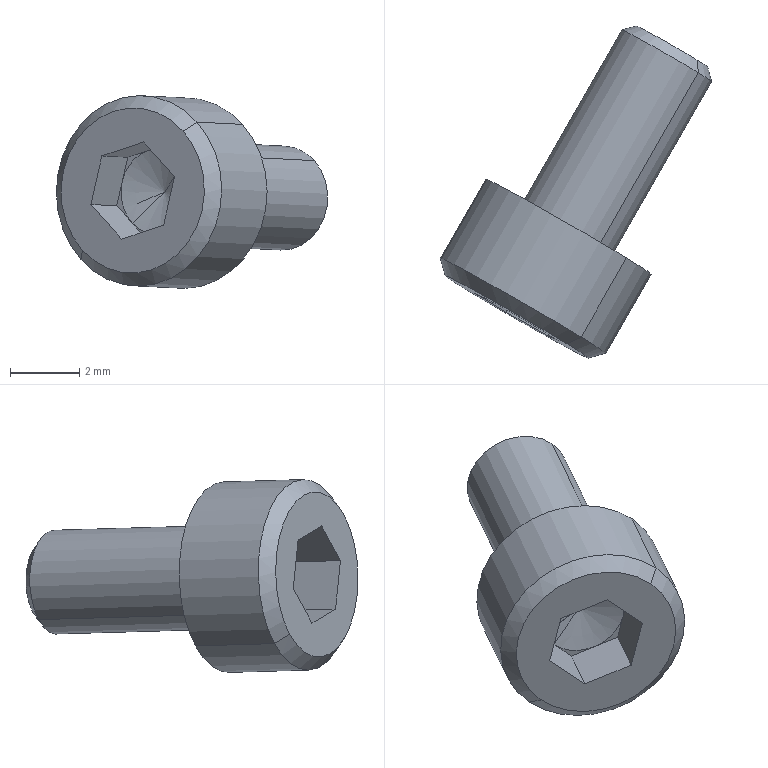Component | SolidWorks | KKSwitch-0710z0-123-1_CB3-6-0710z0-123-14 | 1 solid | 25 faces | box 7.83 x 9.58 x 5.56 mm | volume 103 mm3 | plane 15 | cone 6 | cylinder 4 | commonest cylinder face diameters 3 x2 5.5 x2
STEP:
#1=COLOUR_RGB('',0.7922,0.8196,0.9333);
#2=FILL_AREA_STYLE_COLOUR('',#1);
#3=FILL_AREA_STYLE('',(#2));
#4=SURFACE_STYLE_FILL_AREA(#3);
#5=SURFACE_SIDE_STYLE('',(#4));
#6=SURFACE_STYLE_USAGE(.BOTH.,#5);
#7=PRESENTATION_STYLE_ASSIGNMENT((#6));
#8=CARTESIAN_POINT('',(3.361,-1.018,8.462));
#9=VERTEX_POINT('',#8);
#10=CARTESIAN_POINT('',(3.433,-1.057,8.547));
#11=VERTEX_POINT('',#10);
#12=CARTESIAN_POINT('',(3.397,-1.037,8.504));
#13=DIRECTION('',(0.4977,0.867,-0.02519));
#14=DIRECTION('',(-0.6092,0.3288,-0.7216));
#15=AXIS2_PLACEMENT_3D('',#12,#13,#14);
#16=CIRCLE('',#15,0.05906);
#17=EDGE_CURVE('',#9,#11,#16,.T.);
#18=ORIENTED_EDGE('',*,*,#17,.T.);
#19=CARTESIAN_POINT('',(3.545,-0.8624,8.541));
#20=VERTEX_POINT('',#19);
#21=CARTESIAN_POINT('',(3.489,-0.9595,8.544));
#22=DIRECTION('',(0.4977,0.867,-0.02519));
#23=VECTOR('',#22,39.37);
#24=LINE('',#21,#23);
#25=EDGE_CURVE('',#11,#20,#24,.T.);
#26=ORIENTED_EDGE('',*,*,#25,.T.);
#27=CARTESIAN_POINT('',(3.473,-0.8236,8.456));
#28=VERTEX_POINT('',#27);
#29=CARTESIAN_POINT('',(3.509,-0.843,8.499));
#30=DIRECTION('',(-0.4977,-0.867,0.02519));
#31=DIRECTION('',(-0.6092,0.3288,-0.7216));
#32=AXIS2_PLACEMENT_3D('',#29,#30,#31);
#33=CIRCLE('',#32,0.05906);
#34=EDGE_CURVE('',#20,#28,#33,.T.);
#35=ORIENTED_EDGE('',*,*,#34,.T.);
#36=CARTESIAN_POINT('',(3.417,-0.9207,8.459));
#37=DIRECTION('',(0.4977,0.867,-0.02519));
#38=VECTOR('',#37,39.37);
#39=LINE('',#36,#38);
#40=EDGE_CURVE('',#9,#28,#39,.T.);
#41=ORIENTED_EDGE('',*,*,#40,.F.);
#42=EDGE_LOOP('',(#18,#26,#35,#41));
#43=FACE_OUTER_BOUND('',#42,.T.);
#44=CARTESIAN_POINT('',(3.453,-0.9401,8.501));
#45=DIRECTION('',(0.4977,0.867,-0.02519));
#46=DIRECTION('',(-0.6092,0.3288,-0.7216));
#47=AXIS2_PLACEMENT_3D('',#44,#45,#46);
#48=CYLINDRICAL_SURFACE('',#47,0.05906);
#49=ADVANCED_FACE('',(#43),#48,.T.);
#50=CARTESIAN_POINT('',(3.543,-0.8479,8.532));
#51=VERTEX_POINT('',#50);
#52=CARTESIAN_POINT('',(3.486,-0.817,8.464));
#53=VERTEX_POINT('',#52);
#54=CARTESIAN_POINT('',(3.515,-0.8325,8.498));
#55=DIRECTION('',(-0.4977,-0.867,0.02519));
#56=DIRECTION('',(0.6092,-0.3288,0.7216));
#57=AXIS2_PLACEMENT_3D('',#54,#55,#56);
#58=CIRCLE('',#57,0.04696);
#59=EDGE_CURVE('',#51,#53,#58,.T.);
#60=ORIENTED_EDGE('',*,*,#59,.T.);
#61=CARTESIAN_POINT('',(3.473,-0.8236,8.456));
#62=DIRECTION('',(-0.7827,-0.3806,-0.4924));
#63=VECTOR('',#62,39.37);
#64=LINE('',#61,#63);
#65=EDGE_CURVE('',#53,#28,#64,.T.);
#66=ORIENTED_EDGE('',*,*,#65,.T.);
#67=ORIENTED_EDGE('',*,*,#34,.F.);
#68=CARTESIAN_POINT('',(3.545,-0.8624,8.541));
#69=DIRECTION('',(0.07887,-0.8455,0.5281));
#70=VECTOR('',#69,39.37);
#71=LINE('',#68,#70);
#72=EDGE_CURVE('',#51,#20,#71,.T.);
#73=ORIENTED_EDGE('',*,*,#72,.F.);
#74=EDGE_LOOP('',(#60,#66,#67,#73));
#75=FACE_OUTER_BOUND('',#74,.T.);
#76=CARTESIAN_POINT('',(3.509,-0.843,8.499));
#77=DIRECTION('',(-0.4977,-0.867,0.02519));
#78=DIRECTION('',(0.6092,-0.3288,0.7216));
#79=AXIS2_PLACEMENT_3D('',#76,#77,#78);
#80=CONICAL_SURFACE('',#79,0.05906,0.7854);
#81=ADVANCED_FACE('',(#75),#80,.T.);
#82=CARTESIAN_POINT('',(3.279,-1.092,8.429));
#83=VERTEX_POINT('',#82);
#84=CARTESIAN_POINT('',(3.411,-1.163,8.585));
#85=VERTEX_POINT('',#84);
#86=CARTESIAN_POINT('',(3.345,-1.127,8.507));
#87=DIRECTION('',(0.4977,0.867,-0.02519));
#88=DIRECTION('',(-0.6092,0.3288,-0.7216));
#89=AXIS2_PLACEMENT_3D('',#86,#87,#88);
#90=CIRCLE('',#89,0.1083);
#91=EDGE_CURVE('',#83,#85,#90,.T.);
#92=ORIENTED_EDGE('',*,*,#91,.T.);
#93=CARTESIAN_POINT('',(3.463,-1.073,8.582));
#94=VERTEX_POINT('',#93);
#95=CARTESIAN_POINT('',(3.437,-1.118,8.584));
#96=DIRECTION('',(0.4977,0.867,-0.02519));
#97=VECTOR('',#96,39.37);
#98=LINE('',#95,#97);
#99=EDGE_CURVE('',#85,#94,#98,.T.);
#100=ORIENTED_EDGE('',*,*,#99,.T.);
#101=CARTESIAN_POINT('',(3.331,-1.002,8.426));
#102=VERTEX_POINT('',#101);
#103=CARTESIAN_POINT('',(3.397,-1.037,8.504));
#104=DIRECTION('',(0.4977,0.867,-0.02519));
#105=DIRECTION('',(-0.6092,0.3288,-0.7216));
#106=AXIS2_PLACEMENT_3D('',#103,#104,#105);
#107=CIRCLE('',#106,0.1083);
#108=EDGE_CURVE('',#102,#94,#107,.T.);
#109=ORIENTED_EDGE('',*,*,#108,.F.);
#110=CARTESIAN_POINT('',(3.305,-1.047,8.427));
#111=DIRECTION('',(0.4977,0.867,-0.02519));
#112=VECTOR('',#111,39.37);
#113=LINE('',#110,#112);
#114=EDGE_CURVE('',#83,#102,#113,.T.);
#115=ORIENTED_EDGE('',*,*,#114,.F.);
#116=EDGE_LOOP('',(#92,#100,#109,#115));
#117=FACE_OUTER_BOUND('',#116,.T.);
#118=CARTESIAN_POINT('',(3.371,-1.082,8.505));
#119=DIRECTION('',(0.4977,0.867,-0.02519));
#120=DIRECTION('',(-0.6092,0.3288,-0.7216));
#121=AXIS2_PLACEMENT_3D('',#118,#119,#120);
#122=CYLINDRICAL_SURFACE('',#121,0.1083);
#123=ADVANCED_FACE('',(#117),#122,.T.);
#124=CARTESIAN_POINT('',(3.281,-1.109,8.439));
#125=VERTEX_POINT('',#124);
#126=CARTESIAN_POINT('',(3.395,-1.171,8.575));
#127=VERTEX_POINT('',#126);
#128=CARTESIAN_POINT('',(3.338,-1.14,8.507));
#129=DIRECTION('',(0.4977,0.867,-0.02519));
#130=DIRECTION('',(-0.6092,0.3288,-0.7216));
#131=AXIS2_PLACEMENT_3D('',#128,#129,#130);
#132=CIRCLE('',#131,0.09383);
#133=EDGE_CURVE('',#125,#127,#132,.T.);
#134=ORIENTED_EDGE('',*,*,#133,.T.);
#135=CARTESIAN_POINT('',(3.411,-1.163,8.585));
#136=DIRECTION('',(0.7827,0.3806,0.4924));
#137=VECTOR('',#136,39.37);
#138=LINE('',#135,#137);
#139=EDGE_CURVE('',#127,#85,#138,.T.);
#140=ORIENTED_EDGE('',*,*,#139,.T.);
#141=ORIENTED_EDGE('',*,*,#91,.F.);
#142=CARTESIAN_POINT('',(3.279,-1.092,8.429));
#143=DIRECTION('',(-0.07887,0.8455,-0.5281));
#144=VECTOR('',#143,39.37);
#145=LINE('',#142,#144);
#146=EDGE_CURVE('',#125,#83,#145,.T.);
#147=ORIENTED_EDGE('',*,*,#146,.F.);
#148=EDGE_LOOP('',(#134,#140,#141,#147));
#149=FACE_OUTER_BOUND('',#148,.T.);
#150=CARTESIAN_POINT('',(3.345,-1.127,8.507));
#151=DIRECTION('',(0.4977,0.867,-0.02519));
#152=DIRECTION('',(-0.6092,0.3288,-0.7216));
#153=AXIS2_PLACEMENT_3D('',#150,#151,#152);
#154=CONICAL_SURFACE('',#153,0.1083,0.7854);
#155=ADVANCED_FACE('',(#149),#154,.T.);
#156=CARTESIAN_POINT('',(3.374,-1.077,8.505));
#157=VERTEX_POINT('',#156);
#158=CARTESIAN_POINT('',(3.398,-1.105,8.541));
#159=VERTEX_POINT('',#158);
#160=CARTESIAN_POINT('',(3.398,-1.105,8.541));
#161=DIRECTION('',(0.4597,-0.542,0.7035));
#162=VECTOR('',#161,39.37);
#163=LINE('',#160,#162);
#164=EDGE_CURVE('',#157,#159,#163,.T.);
#165=ORIENTED_EDGE('',*,*,#164,.F.);
#166=CARTESIAN_POINT('',(3.338,-1.072,8.47));
#167=VERTEX_POINT('',#166);
#168=CARTESIAN_POINT('',(3.338,-1.072,8.47));
#169=DIRECTION('',(-0.7173,0.09319,-0.6905));
#170=VECTOR('',#169,39.37);
#171=LINE('',#168,#170);
#172=EDGE_CURVE('',#157,#167,#171,.T.);
#173=ORIENTED_EDGE('',*,*,#172,.T.);
#174=CARTESIAN_POINT('',(3.379,-1.096,8.458));
#175=VERTEX_POINT('',#174);
#176=CARTESIAN_POINT('',(3.368,-1.088,8.506));
#177=DIRECTION('',(-0.4977,-0.867,0.02519));
#178=DIRECTION('',(0.6092,-0.3288,0.7216));
#179=AXIS2_PLACEMENT_3D('',#176,#177,#178);
#180=CIRCLE('',#179,0.04921);
#181=EDGE_CURVE('',#167,#175,#180,.T.);
#182=ORIENTED_EDGE('',*,*,#181,.T.);
#183=CARTESIAN_POINT('',(3.409,-1.113,8.494));
#184=VERTEX_POINT('',#183);
#185=CARTESIAN_POINT('',(3.368,-1.088,8.506));
#186=DIRECTION('',(-0.4977,-0.867,0.02519));
#187=DIRECTION('',(0.6092,-0.3288,0.7216));
#188=AXIS2_PLACEMENT_3D('',#185,#186,#187);
#189=CIRCLE('',#188,0.04921);
#190=EDGE_CURVE('',#175,#184,#189,.T.);
#191=ORIENTED_EDGE('',*,*,#190,.T.);
#192=CARTESIAN_POINT('',(3.368,-1.088,8.506));
#193=DIRECTION('',(-0.4977,-0.867,0.02519));
#194=DIRECTION('',(0.6092,-0.3288,0.7216));
#195=AXIS2_PLACEMENT_3D('',#192,#193,#194);
#196=CIRCLE('',#195,0.04921);
#197=EDGE_CURVE('',#184,#159,#196,.T.);
#198=ORIENTED_EDGE('',*,*,#197,.T.);
#199=EDGE_LOOP('',(#165,#173,#182,#191,#198));
#200=FACE_OUTER_BOUND('',#199,.T.);
#201=CARTESIAN_POINT('',(3.368,-1.088,8.506));
#202=DIRECTION('',(-0.4977,-0.867,0.02519));
#203=DIRECTION('',(0.6092,-0.3288,0.7216));
#204=AXIS2_PLACEMENT_3D('',#201,#202,#203);
#205=CONICAL_SURFACE('',#204,0.04921,1.309);
#206=ADVANCED_FACE('',(#200),#205,.F.);
#207=ORIENTED_EDGE('',*,*,#25,.F.);
#208=CARTESIAN_POINT('',(3.397,-1.037,8.504));
#209=DIRECTION('',(0.4977,0.867,-0.02519));
#210=DIRECTION('',(-0.6092,0.3288,-0.7216));
#211=AXIS2_PLACEMENT_3D('',#208,#209,#210);
#212=CIRCLE('',#211,0.05906);
#213=EDGE_CURVE('',#11,#9,#212,.T.);
#214=ORIENTED_EDGE('',*,*,#213,.T.);
#215=ORIENTED_EDGE('',*,*,#40,.T.);
#216=CARTESIAN_POINT('',(3.509,-0.843,8.499));
#217=DIRECTION('',(-0.4977,-0.867,0.02519));
#218=DIRECTION('',(-0.6092,0.3288,-0.7216));
#219=AXIS2_PLACEMENT_3D('',#216,#217,#218);
#220=CIRCLE('',#219,0.05906);
#221=EDGE_CURVE('',#28,#20,#220,.T.);
#222=ORIENTED_EDGE('',*,*,#221,.T.);
#223=EDGE_LOOP('',(#207,#214,#215,#222));
#224=FACE_OUTER_BOUND('',#223,.T.);
#225=CARTESIAN_POINT('',(3.453,-0.9401,8.501));
#226=DIRECTION('',(0.4977,0.867,-0.02519));
#227=DIRECTION('',(-0.6092,0.3288,-0.7216));
#228=AXIS2_PLACEMENT_3D('',#225,#226,#227);
#229=CYLINDRICAL_SURFACE('',#228,0.05906);
#230=ADVANCED_FACE('',(#224),#229,.T.);
#231=ORIENTED_EDGE('',*,*,#17,.F.);
#232=ORIENTED_EDGE('',*,*,#213,.F.);
#233=EDGE_LOOP('',(#231,#232));
#234=FACE_BOUND('',#233,.T.);
#235=ORIENTED_EDGE('',*,*,#108,.T.);
#236=CARTESIAN_POINT('',(3.397,-1.037,8.504));
#237=DIRECTION('',(0.4977,0.867,-0.02519));
#238=DIRECTION('',(-0.6092,0.3288,-0.7216));
#239=AXIS2_PLACEMENT_3D('',#236,#237,#238);
#240=CIRCLE('',#239,0.1083);
#241=EDGE_CURVE('',#94,#102,#240,.T.);
#242=ORIENTED_EDGE('',*,*,#241,.T.);
#243=EDGE_LOOP('',(#235,#242));
#244=FACE_OUTER_BOUND('',#243,.T.);
#245=CARTESIAN_POINT('',(3.345,-1.006,8.562));
#246=DIRECTION('',(0.4977,0.867,-0.02519));
#247=DIRECTION('',(-0.6092,0.3288,-0.7216));
#248=AXIS2_PLACEMENT_3D('',#245,#246,#247);
#249=PLANE('',#248);
#250=ADVANCED_FACE('',(#234,#244),#249,.T.);
#251=ORIENTED_EDGE('',*,*,#65,.F.);
#252=CARTESIAN_POINT('',(3.515,-0.8325,8.498));
#253=DIRECTION('',(-0.4977,-0.867,0.02519));
#254=DIRECTION('',(0.6092,-0.3288,0.7216));
#255=AXIS2_PLACEMENT_3D('',#252,#253,#254);
#256=CIRCLE('',#255,0.04696);
#257=EDGE_CURVE('',#53,#51,#256,.T.);
#258=ORIENTED_EDGE('',*,*,#257,.T.);
#259=ORIENTED_EDGE('',*,*,#72,.T.);
#260=ORIENTED_EDGE('',*,*,#221,.F.);
#261=EDGE_LOOP('',(#251,#258,#259,#260));
#262=FACE_OUTER_BOUND('',#261,.T.);
#263=CARTESIAN_POINT('',(3.509,-0.843,8.499));
#264=DIRECTION('',(-0.4977,-0.867,0.02519));
#265=DIRECTION('',(0.6092,-0.3288,0.7216));
#266=AXIS2_PLACEMENT_3D('',#263,#264,#265);
#267=CONICAL_SURFACE('',#266,0.05906,0.7854);
#268=ADVANCED_FACE('',(#262),#267,.T.);
#269=ORIENTED_EDGE('',*,*,#99,.F.);
#270=CARTESIAN_POINT('',(3.345,-1.127,8.507));
#271=DIRECTION('',(0.4977,0.867,-0.02519));
#272=DIRECTION('',(-0.6092,0.3288,-0.7216));
#273=AXIS2_PLACEMENT_3D('',#270,#271,#272);
#274=CIRCLE('',#273,0.1083);
#275=EDGE_CURVE('',#85,#83,#274,.T.);
#276=ORIENTED_EDGE('',*,*,#275,.T.);
#277=ORIENTED_EDGE('',*,*,#114,.T.);
#278=ORIENTED_EDGE('',*,*,#241,.F.);
#279=EDGE_LOOP('',(#269,#276,#277,#278));
#280=FACE_OUTER_BOUND('',#279,.T.);
#281=CARTESIAN_POINT('',(3.371,-1.082,8.505));
#282=DIRECTION('',(0.4977,0.867,-0.02519));
#283=DIRECTION('',(-0.6092,0.3288,-0.7216));
#284=AXIS2_PLACEMENT_3D('',#281,#282,#283);
#285=CYLINDRICAL_SURFACE('',#284,0.1083);
#286=ADVANCED_FACE('',(#280),#285,.T.);
#287=ORIENTED_EDGE('',*,*,#59,.F.);
#288=ORIENTED_EDGE('',*,*,#257,.F.);
#289=EDGE_LOOP('',(#287,#288));
#290=FACE_OUTER_BOUND('',#289,.T.);
#291=CARTESIAN_POINT('',(3.5,-0.8237,8.514));
#292=DIRECTION('',(0.4977,0.867,-0.02519));
#293=DIRECTION('',(-0.6092,0.3288,-0.7216));
#294=AXIS2_PLACEMENT_3D('',#291,#292,#293);
#295=PLANE('',#294);
#296=ADVANCED_FACE('',(#290),#295,.T.);
#297=ORIENTED_EDGE('',*,*,#139,.F.);
#298=CARTESIAN_POINT('',(3.338,-1.14,8.507));
#299=DIRECTION('',(0.4977,0.867,-0.02519));
#300=DIRECTION('',(-0.6092,0.3288,-0.7216));
#301=AXIS2_PLACEMENT_3D('',#298,#299,#300);
#302=CIRCLE('',#301,0.09383);
#303=EDGE_CURVE('',#127,#125,#302,.T.);
#304=ORIENTED_EDGE('',*,*,#303,.T.);
#305=ORIENTED_EDGE('',*,*,#146,.T.);
#306=ORIENTED_EDGE('',*,*,#275,.F.);
#307=EDGE_LOOP('',(#297,#304,#305,#306));
#308=FACE_OUTER_BOUND('',#307,.T.);
#309=CARTESIAN_POINT('',(3.345,-1.127,8.507));
#310=DIRECTION('',(0.4977,0.867,-0.02519));
#311=DIRECTION('',(-0.6092,0.3288,-0.7216));
#312=AXIS2_PLACEMENT_3D('',#309,#310,#311);
#313=CONICAL_SURFACE('',#312,0.1083,0.7854);
#314=ADVANCED_FACE('',(#308),#313,.T.);
#315=ORIENTED_EDGE('',*,*,#133,.F.);
#316=ORIENTED_EDGE('',*,*,#303,.F.);
#317=EDGE_LOOP('',(#315,#316));
#318=FACE_OUTER_BOUND('',#317,.T.);
#319=CARTESIAN_POINT('',(3.291,-1.113,8.491));
#320=VERTEX_POINT('',#319);
#321=CARTESIAN_POINT('',(3.303,-1.118,8.546));
#322=VERTEX_POINT('',#321);
#323=CARTESIAN_POINT('',(3.291,-1.113,8.491));
#324=DIRECTION('',(0.219,-0.09749,0.9709));
#325=VECTOR('',#324,39.37);
#326=LINE('',#323,#325);
#327=EDGE_CURVE('',#320,#322,#326,.T.);
#328=ORIENTED_EDGE('',*,*,#327,.T.);
#329=CARTESIAN_POINT('',(3.351,-1.145,8.562));
#330=VERTEX_POINT('',#329);
#331=CARTESIAN_POINT('',(3.303,-1.118,8.546));
#332=DIRECTION('',(0.8363,-0.472,0.279));
#333=VECTOR('',#332,39.37);
#334=LINE('',#331,#333);
#335=EDGE_CURVE('',#322,#330,#334,.T.);
#336=ORIENTED_EDGE('',*,*,#335,.T.);
#337=CARTESIAN_POINT('',(3.386,-1.167,8.523));
#338=VERTEX_POINT('',#337);
#339=CARTESIAN_POINT('',(3.339,-1.138,8.575));
#340=DIRECTION('',(0.6173,-0.3745,-0.6918));
#341=VECTOR('',#340,39.37);
#342=LINE('',#339,#341);
#343=EDGE_CURVE('',#330,#338,#342,.T.);
#344=ORIENTED_EDGE('',*,*,#343,.T.);
#345=CARTESIAN_POINT('',(3.373,-1.161,8.468));
#346=VERTEX_POINT('',#345);
#347=CARTESIAN_POINT('',(3.386,-1.167,8.523));
#348=DIRECTION('',(-0.219,0.09749,-0.9709));
#349=VECTOR('',#348,39.37);
#350=LINE('',#347,#349);
#351=EDGE_CURVE('',#338,#346,#350,.T.);
#352=ORIENTED_EDGE('',*,*,#351,.T.);
#353=CARTESIAN_POINT('',(3.326,-1.134,8.452));
#354=VERTEX_POINT('',#353);
#355=CARTESIAN_POINT('',(3.373,-1.161,8.468));
#356=DIRECTION('',(-0.8363,0.472,-0.279));
#357=VECTOR('',#356,39.37);
#358=LINE('',#355,#357);
#359=EDGE_CURVE('',#346,#354,#358,.T.);
#360=ORIENTED_EDGE('',*,*,#359,.T.);
#361=CARTESIAN_POINT('',(3.279,-1.106,8.504));
#362=DIRECTION('',(-0.6173,0.3745,0.6918));
#363=VECTOR('',#362,39.37);
#364=LINE('',#361,#363);
#365=EDGE_CURVE('',#354,#320,#364,.T.);
#366=ORIENTED_EDGE('',*,*,#365,.T.);
#367=EDGE_LOOP('',(#328,#336,#344,#352,#360,#366));
#368=FACE_BOUND('',#367,.T.);
#369=CARTESIAN_POINT('',(3.309,-1.122,8.54));
#370=DIRECTION('',(-0.4977,-0.867,0.02519));
#371=DIRECTION('',(0.6092,-0.3288,0.7216));
#372=AXIS2_PLACEMENT_3D('',#369,#370,#371);
#373=PLANE('',#372);
#374=ADVANCED_FACE('',(#318,#368),#373,.T.);
#375=CARTESIAN_POINT('',(3.333,-1.067,8.545));
#376=VERTEX_POINT('',#375);
#377=CARTESIAN_POINT('',(3.303,-1.118,8.546));
#378=DIRECTION('',(-0.4977,-0.867,0.02519));
#379=VECTOR('',#378,39.37);
#380=LINE('',#377,#379);
#381=EDGE_CURVE('',#376,#322,#380,.T.);
#382=ORIENTED_EDGE('',*,*,#381,.F.);
#383=CARTESIAN_POINT('',(3.356,-1.081,8.553));
#384=VERTEX_POINT('',#383);
#385=CARTESIAN_POINT('',(3.38,-1.094,8.561));
#386=DIRECTION('',(-0.8363,0.472,-0.279));
#387=VECTOR('',#386,39.37);
#388=LINE('',#385,#387);
#389=EDGE_CURVE('',#384,#376,#388,.T.);
#390=ORIENTED_EDGE('',*,*,#389,.F.);
#391=CARTESIAN_POINT('',(3.38,-1.094,8.561));
#392=VERTEX_POINT('',#391);
#393=CARTESIAN_POINT('',(3.38,-1.094,8.561));
#394=DIRECTION('',(-0.8363,0.472,-0.279));
#395=VECTOR('',#394,39.37);
#396=LINE('',#393,#395);
#397=EDGE_CURVE('',#392,#384,#396,.T.);
#398=ORIENTED_EDGE('',*,*,#397,.F.);
#399=CARTESIAN_POINT('',(3.351,-1.145,8.562));
#400=DIRECTION('',(0.4977,0.867,-0.02519));
#401=VECTOR('',#400,39.37);
#402=LINE('',#399,#401);
#403=EDGE_CURVE('',#330,#392,#402,.T.);
#404=ORIENTED_EDGE('',*,*,#403,.F.);
#405=ORIENTED_EDGE('',*,*,#335,.F.);
#406=EDGE_LOOP('',(#382,#390,#398,#404,#405));
#407=FACE_OUTER_BOUND('',#406,.T.);
#408=CARTESIAN_POINT('',(3.351,-1.145,8.562));
#409=DIRECTION('',(-0.23,0.1599,0.96));
#410=DIRECTION('',(0.8363,-0.472,0.279));
#411=AXIS2_PLACEMENT_3D('',#408,#409,#410);
#412=PLANE('',#411);
#413=ADVANCED_FACE('',(#407),#412,.F.);
#414=CARTESIAN_POINT('',(3.32,-1.062,8.49));
#415=VERTEX_POINT('',#414);
#416=CARTESIAN_POINT('',(3.291,-1.113,8.491));
#417=DIRECTION('',(-0.4977,-0.867,0.02519));
#418=VECTOR('',#417,39.37);
#419=LINE('',#416,#418);
#420=EDGE_CURVE('',#415,#320,#419,.T.);
#421=ORIENTED_EDGE('',*,*,#420,.F.);
#422=CARTESIAN_POINT('',(3.326,-1.064,8.517));
#423=VERTEX_POINT('',#422);
#424=CARTESIAN_POINT('',(3.333,-1.067,8.545));
#425=DIRECTION('',(-0.219,0.09749,-0.9709));
#426=VECTOR('',#425,39.37);
#427=LINE('',#424,#426);
#428=EDGE_CURVE('',#423,#415,#427,.T.);
#429=ORIENTED_EDGE('',*,*,#428,.F.);
#430=CARTESIAN_POINT('',(3.333,-1.067,8.545));
#431=DIRECTION('',(-0.219,0.09749,-0.9709));
#432=VECTOR('',#431,39.37);
#433=LINE('',#430,#432);
#434=EDGE_CURVE('',#376,#423,#433,.T.);
#435=ORIENTED_EDGE('',*,*,#434,.F.);
#436=ORIENTED_EDGE('',*,*,#381,.T.);
#437=ORIENTED_EDGE('',*,*,#327,.F.);
#438=EDGE_LOOP('',(#421,#429,#435,#436,#437));
#439=FACE_OUTER_BOUND('',#438,.T.);
#440=CARTESIAN_POINT('',(3.303,-1.118,8.546));
#441=DIRECTION('',(-0.8393,0.4887,0.2383));
#442=DIRECTION('',(0.219,-0.09749,0.9709));
#443=AXIS2_PLACEMENT_3D('',#440,#441,#442);
#444=PLANE('',#443);
#445=ADVANCED_FACE('',(#439),#444,.F.);
#446=CARTESIAN_POINT('',(3.355,-1.083,8.45));
#447=VERTEX_POINT('',#446);
#448=CARTESIAN_POINT('',(3.326,-1.134,8.452));
#449=DIRECTION('',(-0.4977,-0.867,0.02519));
#450=VECTOR('',#449,39.37);
#451=LINE('',#448,#450);
#452=EDGE_CURVE('',#447,#354,#451,.T.);
#453=ORIENTED_EDGE('',*,*,#452,.F.);
#454=CARTESIAN_POINT('',(3.32,-1.062,8.49));
#455=DIRECTION('',(0.6173,-0.3745,-0.6918));
#456=VECTOR('',#455,39.37);
#457=LINE('',#454,#456);
#458=EDGE_CURVE('',#167,#447,#457,.T.);
#459=ORIENTED_EDGE('',*,*,#458,.F.);
#460=CARTESIAN_POINT('',(3.32,-1.062,8.49));
#461=DIRECTION('',(0.6173,-0.3745,-0.6918));
#462=VECTOR('',#461,39.37);
#463=LINE('',#460,#462);
#464=EDGE_CURVE('',#415,#167,#463,.T.);
#465=ORIENTED_EDGE('',*,*,#464,.F.);
#466=ORIENTED_EDGE('',*,*,#420,.T.);
#467=ORIENTED_EDGE('',*,*,#365,.F.);
#468=EDGE_LOOP('',(#453,#459,#465,#466,#467));
#469=FACE_OUTER_BOUND('',#468,.T.);
#470=CARTESIAN_POINT('',(3.291,-1.113,8.491));
#471=DIRECTION('',(-0.6092,0.3288,-0.7216));
#472=DIRECTION('',(-0.4977,-0.867,0.02519));
#473=AXIS2_PLACEMENT_3D('',#470,#471,#472);
#474=PLANE('',#473);
#475=ADVANCED_FACE('',(#469),#474,.F.);
#476=CARTESIAN_POINT('',(3.403,-1.11,8.466));
#477=VERTEX_POINT('',#476);
#478=CARTESIAN_POINT('',(3.373,-1.161,8.468));
#479=DIRECTION('',(-0.4977,-0.867,0.02519));
#480=VECTOR('',#479,39.37);
#481=LINE('',#478,#480);
#482=EDGE_CURVE('',#477,#346,#481,.T.);
#483=ORIENTED_EDGE('',*,*,#482,.F.);
#484=CARTESIAN_POINT('',(3.355,-1.083,8.45));
#485=DIRECTION('',(0.8363,-0.472,0.279));
#486=VECTOR('',#485,39.37);
#487=LINE('',#484,#486);
#488=EDGE_CURVE('',#175,#477,#487,.T.);
#489=ORIENTED_EDGE('',*,*,#488,.F.);
#490=CARTESIAN_POINT('',(3.355,-1.083,8.45));
#491=DIRECTION('',(0.8363,-0.472,0.279));
#492=VECTOR('',#491,39.37);
#493=LINE('',#490,#492);
#494=EDGE_CURVE('',#447,#175,#493,.T.);
#495=ORIENTED_EDGE('',*,*,#494,.F.);
#496=ORIENTED_EDGE('',*,*,#452,.T.);
#497=ORIENTED_EDGE('',*,*,#359,.F.);
#498=EDGE_LOOP('',(#483,#489,#495,#496,#497));
#499=FACE_OUTER_BOUND('',#498,.T.);
#500=CARTESIAN_POINT('',(3.326,-1.134,8.452));
#501=DIRECTION('',(0.23,-0.1599,-0.96));
#502=DIRECTION('',(-0.8363,0.472,-0.279));
#503=AXIS2_PLACEMENT_3D('',#500,#501,#502);
#504=PLANE('',#503);
#505=ADVANCED_FACE('',(#499),#504,.F.);
#506=CARTESIAN_POINT('',(3.415,-1.115,8.521));
#507=VERTEX_POINT('',#506);
#508=CARTESIAN_POINT('',(3.386,-1.167,8.523));
#509=DIRECTION('',(-0.4977,-0.867,0.02519));
#510=VECTOR('',#509,39.37);
#511=LINE('',#508,#510);
#512=EDGE_CURVE('',#507,#338,#511,.T.);
#513=ORIENTED_EDGE('',*,*,#512,.F.);
#514=CARTESIAN_POINT('',(3.403,-1.11,8.466));
#515=DIRECTION('',(0.219,-0.09749,0.9709));
#516=VECTOR('',#515,39.37);
#517=LINE('',#514,#516);
#518=EDGE_CURVE('',#184,#507,#517,.T.);
#519=ORIENTED_EDGE('',*,*,#518,.F.);
#520=CARTESIAN_POINT('',(3.403,-1.11,8.466));
#521=DIRECTION('',(0.219,-0.09749,0.9709));
#522=VECTOR('',#521,39.37);
#523=LINE('',#520,#522);
#524=EDGE_CURVE('',#477,#184,#523,.T.);
#525=ORIENTED_EDGE('',*,*,#524,.F.);
#526=ORIENTED_EDGE('',*,*,#482,.T.);
#527=ORIENTED_EDGE('',*,*,#351,.F.);
#528=EDGE_LOOP('',(#513,#519,#525,#526,#527));
#529=FACE_OUTER_BOUND('',#528,.T.);
#530=CARTESIAN_POINT('',(3.373,-1.161,8.468));
#531=DIRECTION('',(0.8393,-0.4887,-0.2383));
#532=DIRECTION('',(-0.219,0.09749,-0.9709));
#533=AXIS2_PLACEMENT_3D('',#530,#531,#532);
#534=PLANE('',#533);
#535=ADVANCED_FACE('',(#529),#534,.F.);
#536=ORIENTED_EDGE('',*,*,#403,.T.);
#537=CARTESIAN_POINT('',(3.415,-1.115,8.521));
#538=DIRECTION('',(-0.6173,0.3745,0.6918));
#539=VECTOR('',#538,39.37);
#540=LINE('',#537,#539);
#541=EDGE_CURVE('',#159,#392,#540,.T.);
#542=ORIENTED_EDGE('',*,*,#541,.F.);
#543=CARTESIAN_POINT('',(3.415,-1.115,8.521));
#544=DIRECTION('',(-0.6173,0.3745,0.6918));
#545=VECTOR('',#544,39.37);
#546=LINE('',#543,#545);
#547=EDGE_CURVE('',#507,#159,#546,.T.);
#548=ORIENTED_EDGE('',*,*,#547,.F.);
#549=ORIENTED_EDGE('',*,*,#512,.T.);
#550=ORIENTED_EDGE('',*,*,#343,.F.);
#551=EDGE_LOOP('',(#536,#542,#548,#549,#550));
#552=FACE_OUTER_BOUND('',#551,.T.);
#553=CARTESIAN_POINT('',(3.386,-1.167,8.523));
#554=DIRECTION('',(0.6092,-0.3288,0.7216));
#555=DIRECTION('',(0.4977,0.867,-0.02519));
#556=AXIS2_PLACEMENT_3D('',#553,#554,#555);
#557=PLANE('',#556);
#558=ADVANCED_FACE('',(#552),#557,.F.);
#559=ORIENTED_EDGE('',*,*,#389,.T.);
#560=ORIENTED_EDGE('',*,*,#434,.T.);
#561=CARTESIAN_POINT('',(3.368,-1.088,8.506));
#562=DIRECTION('',(-0.4977,-0.867,0.02519));
#563=DIRECTION('',(0.6092,-0.3288,0.7216));
#564=AXIS2_PLACEMENT_3D('',#561,#562,#563);
#565=CIRCLE('',#564,0.04921);
#566=EDGE_CURVE('',#384,#423,#565,.T.);
#567=ORIENTED_EDGE('',*,*,#566,.F.);
#568=EDGE_LOOP('',(#559,#560,#567));
#569=FACE_OUTER_BOUND('',#568,.T.);
#570=CARTESIAN_POINT('',(3.368,-1.088,8.506));
#571=DIRECTION('',(0.4977,0.867,-0.02519));
#572=DIRECTION('',(-0.6092,0.3288,-0.7216));
#573=AXIS2_PLACEMENT_3D('',#570,#571,#572);
#574=PLANE('',#573);
#575=ADVANCED_FACE('',(#569),#574,.F.);
#576=ORIENTED_EDGE('',*,*,#541,.T.);
#577=ORIENTED_EDGE('',*,*,#397,.T.);
#578=CARTESIAN_POINT('',(3.368,-1.088,8.506));
#579=DIRECTION('',(-0.4977,-0.867,0.02519));
#580=DIRECTION('',(0.6092,-0.3288,0.7216));
#581=AXIS2_PLACEMENT_3D('',#578,#579,#580);
#582=CIRCLE('',#581,0.04921);
#583=EDGE_CURVE('',#159,#384,#582,.T.);
#584=ORIENTED_EDGE('',*,*,#583,.F.);
#585=EDGE_LOOP('',(#576,#577,#584));
#586=FACE_OUTER_BOUND('',#585,.T.);
#587=CARTESIAN_POINT('',(3.368,-1.088,8.506));
#588=DIRECTION('',(0.4977,0.867,-0.02519));
#589=DIRECTION('',(-0.6092,0.3288,-0.7216));
#590=AXIS2_PLACEMENT_3D('',#587,#588,#589);
#591=PLANE('',#590);
#592=ADVANCED_FACE('',(#586),#591,.F.);
#593=ORIENTED_EDGE('',*,*,#428,.T.);
#594=ORIENTED_EDGE('',*,*,#464,.T.);
#595=CARTESIAN_POINT('',(3.368,-1.088,8.506));
#596=DIRECTION('',(-0.4977,-0.867,0.02519));
#597=DIRECTION('',(0.6092,-0.3288,0.7216));
#598=AXIS2_PLACEMENT_3D('',#595,#596,#597);
#599=CIRCLE('',#598,0.04921);
#600=EDGE_CURVE('',#423,#167,#599,.T.);
#601=ORIENTED_EDGE('',*,*,#600,.F.);
#602=EDGE_LOOP('',(#593,#594,#601));
#603=FACE_OUTER_BOUND('',#602,.T.);
#604=CARTESIAN_POINT('',(3.368,-1.088,8.506));
#605=DIRECTION('',(0.4977,0.867,-0.02519));
#606=DIRECTION('',(-0.6092,0.3288,-0.7216));
#607=AXIS2_PLACEMENT_3D('',#604,#605,#606);
#608=PLANE('',#607);
#609=ADVANCED_FACE('',(#603),#608,.F.);
#610=ORIENTED_EDGE('',*,*,#458,.T.);
#611=ORIENTED_EDGE('',*,*,#494,.T.);
#612=ORIENTED_EDGE('',*,*,#181,.F.);
#613=EDGE_LOOP('',(#610,#611,#612));
#614=FACE_OUTER_BOUND('',#613,.T.);
#615=CARTESIAN_POINT('',(3.368,-1.088,8.506));
#616=DIRECTION('',(0.4977,0.867,-0.02519));
#617=DIRECTION('',(-0.6092,0.3288,-0.7216));
#618=AXIS2_PLACEMENT_3D('',#615,#616,#617);
#619=PLANE('',#618);
#620=ADVANCED_FACE('',(#614),#619,.F.);
#621=ORIENTED_EDGE('',*,*,#488,.T.);
#622=ORIENTED_EDGE('',*,*,#524,.T.);
#623=ORIENTED_EDGE('',*,*,#190,.F.);
#624=EDGE_LOOP('',(#621,#622,#623));
#625=FACE_OUTER_BOUND('',#624,.T.);
#626=CARTESIAN_POINT('',(3.368,-1.088,8.506));
#627=DIRECTION('',(0.4977,0.867,-0.02519));
#628=DIRECTION('',(-0.6092,0.3288,-0.7216));
#629=AXIS2_PLACEMENT_3D('',#626,#627,#628);
#630=PLANE('',#629);
#631=ADVANCED_FACE('',(#625),#630,.F.);
#632=ORIENTED_EDGE('',*,*,#518,.T.);
#633=ORIENTED_EDGE('',*,*,#547,.T.);
#634=ORIENTED_EDGE('',*,*,#197,.F.);
#635=EDGE_LOOP('',(#632,#633,#634));
#636=FACE_OUTER_BOUND('',#635,.T.);
#637=CARTESIAN_POINT('',(3.368,-1.088,8.506));
#638=DIRECTION('',(0.4977,0.867,-0.02519));
#639=DIRECTION('',(-0.6092,0.3288,-0.7216));
#640=AXIS2_PLACEMENT_3D('',#637,#638,#639);
#641=PLANE('',#640);
#642=ADVANCED_FACE('',(#636),#641,.F.);
#643=ORIENTED_EDGE('',*,*,#172,.F.);
#644=ORIENTED_EDGE('',*,*,#164,.T.);
#645=ORIENTED_EDGE('',*,*,#583,.T.);
#646=ORIENTED_EDGE('',*,*,#566,.T.);
#647=ORIENTED_EDGE('',*,*,#600,.T.);
#648=EDGE_LOOP('',(#643,#644,#645,#646,#647));
#649=FACE_OUTER_BOUND('',#648,.T.);
#650=CARTESIAN_POINT('',(3.368,-1.088,8.506));
#651=DIRECTION('',(-0.4977,-0.867,0.02519));
#652=DIRECTION('',(0.6092,-0.3288,0.7216));
#653=AXIS2_PLACEMENT_3D('',#650,#651,#652);
#654=CONICAL_SURFACE('',#653,0.04921,1.309);
#655=ADVANCED_FACE('',(#649),#654,.F.);
#656=CLOSED_SHELL('',(#49,#81,#123,#155,#206,#230,#250,#268,#286,#296,#314,#374,#413,#445,#475,#505,#535,#558,#575,#592,#609,#620,#631,#642,#655));
#657=MANIFOLD_SOLID_BREP('',#656);
#658=STYLED_ITEM('',(#7),#657);
#659=(LENGTH_UNIT()NAMED_UNIT(*)SI_UNIT($,.METRE.));
#660=LENGTH_MEASURE_WITH_UNIT(LENGTH_MEASURE(0.0254),#659);
#661=DIMENSIONAL_EXPONENTS(1.,0.,0.,0.,0.,0.,0.);
#662=(CONVERSION_BASED_UNIT('',#660)LENGTH_UNIT()NAMED_UNIT(#661));
#663=UNCERTAINTY_MEASURE_WITH_UNIT(LENGTH_MEASURE(0.00001),#662,'','');
#664=(NAMED_UNIT(*)PLANE_ANGLE_UNIT()SI_UNIT($,.RADIAN.));
#665=(NAMED_UNIT(*)SI_UNIT($,.STERADIAN.)SOLID_ANGLE_UNIT());
#666=(GEOMETRIC_REPRESENTATION_CONTEXT(3)GLOBAL_UNCERTAINTY_ASSIGNED_CONTEXT((#663))GLOBAL_UNIT_ASSIGNED_CONTEXT((#662,#664,#665))REPRESENTATION_CONTEXT('',''));
#667=MECHANICAL_DESIGN_GEOMETRIC_PRESENTATION_REPRESENTATION('',(#658),#666);
#668=PRESENTATION_LAYER_ASSIGNMENT('','',(#658));
#669=CARTESIAN_POINT('',(0.,0.,0.));
#670=DIRECTION('',(0.,0.,1.));
#671=DIRECTION('',(1.,0.,0.));
#672=AXIS2_PLACEMENT_3D('',#669,#670,#671);
#673=(LENGTH_UNIT()NAMED_UNIT(*)SI_UNIT($,.METRE.));
#674=LENGTH_MEASURE_WITH_UNIT(LENGTH_MEASURE(0.0254),#673);
#675=DIMENSIONAL_EXPONENTS(1.,0.,0.,0.,0.,0.,0.);
#676=(CONVERSION_BASED_UNIT('',#674)LENGTH_UNIT()NAMED_UNIT(#675));
#677=UNCERTAINTY_MEASURE_WITH_UNIT(LENGTH_MEASURE(0.00001),#676,'','');
#678=(NAMED_UNIT(*)PLANE_ANGLE_UNIT()SI_UNIT($,.RADIAN.));
#679=(NAMED_UNIT(*)SI_UNIT($,.STERADIAN.)SOLID_ANGLE_UNIT());
#680=(GEOMETRIC_REPRESENTATION_CONTEXT(3)GLOBAL_UNCERTAINTY_ASSIGNED_CONTEXT((#677))GLOBAL_UNIT_ASSIGNED_CONTEXT((#676,#678,#679))REPRESENTATION_CONTEXT('',''));
#681=ADVANCED_BREP_SHAPE_REPRESENTATION('',(#657,#672),#680);